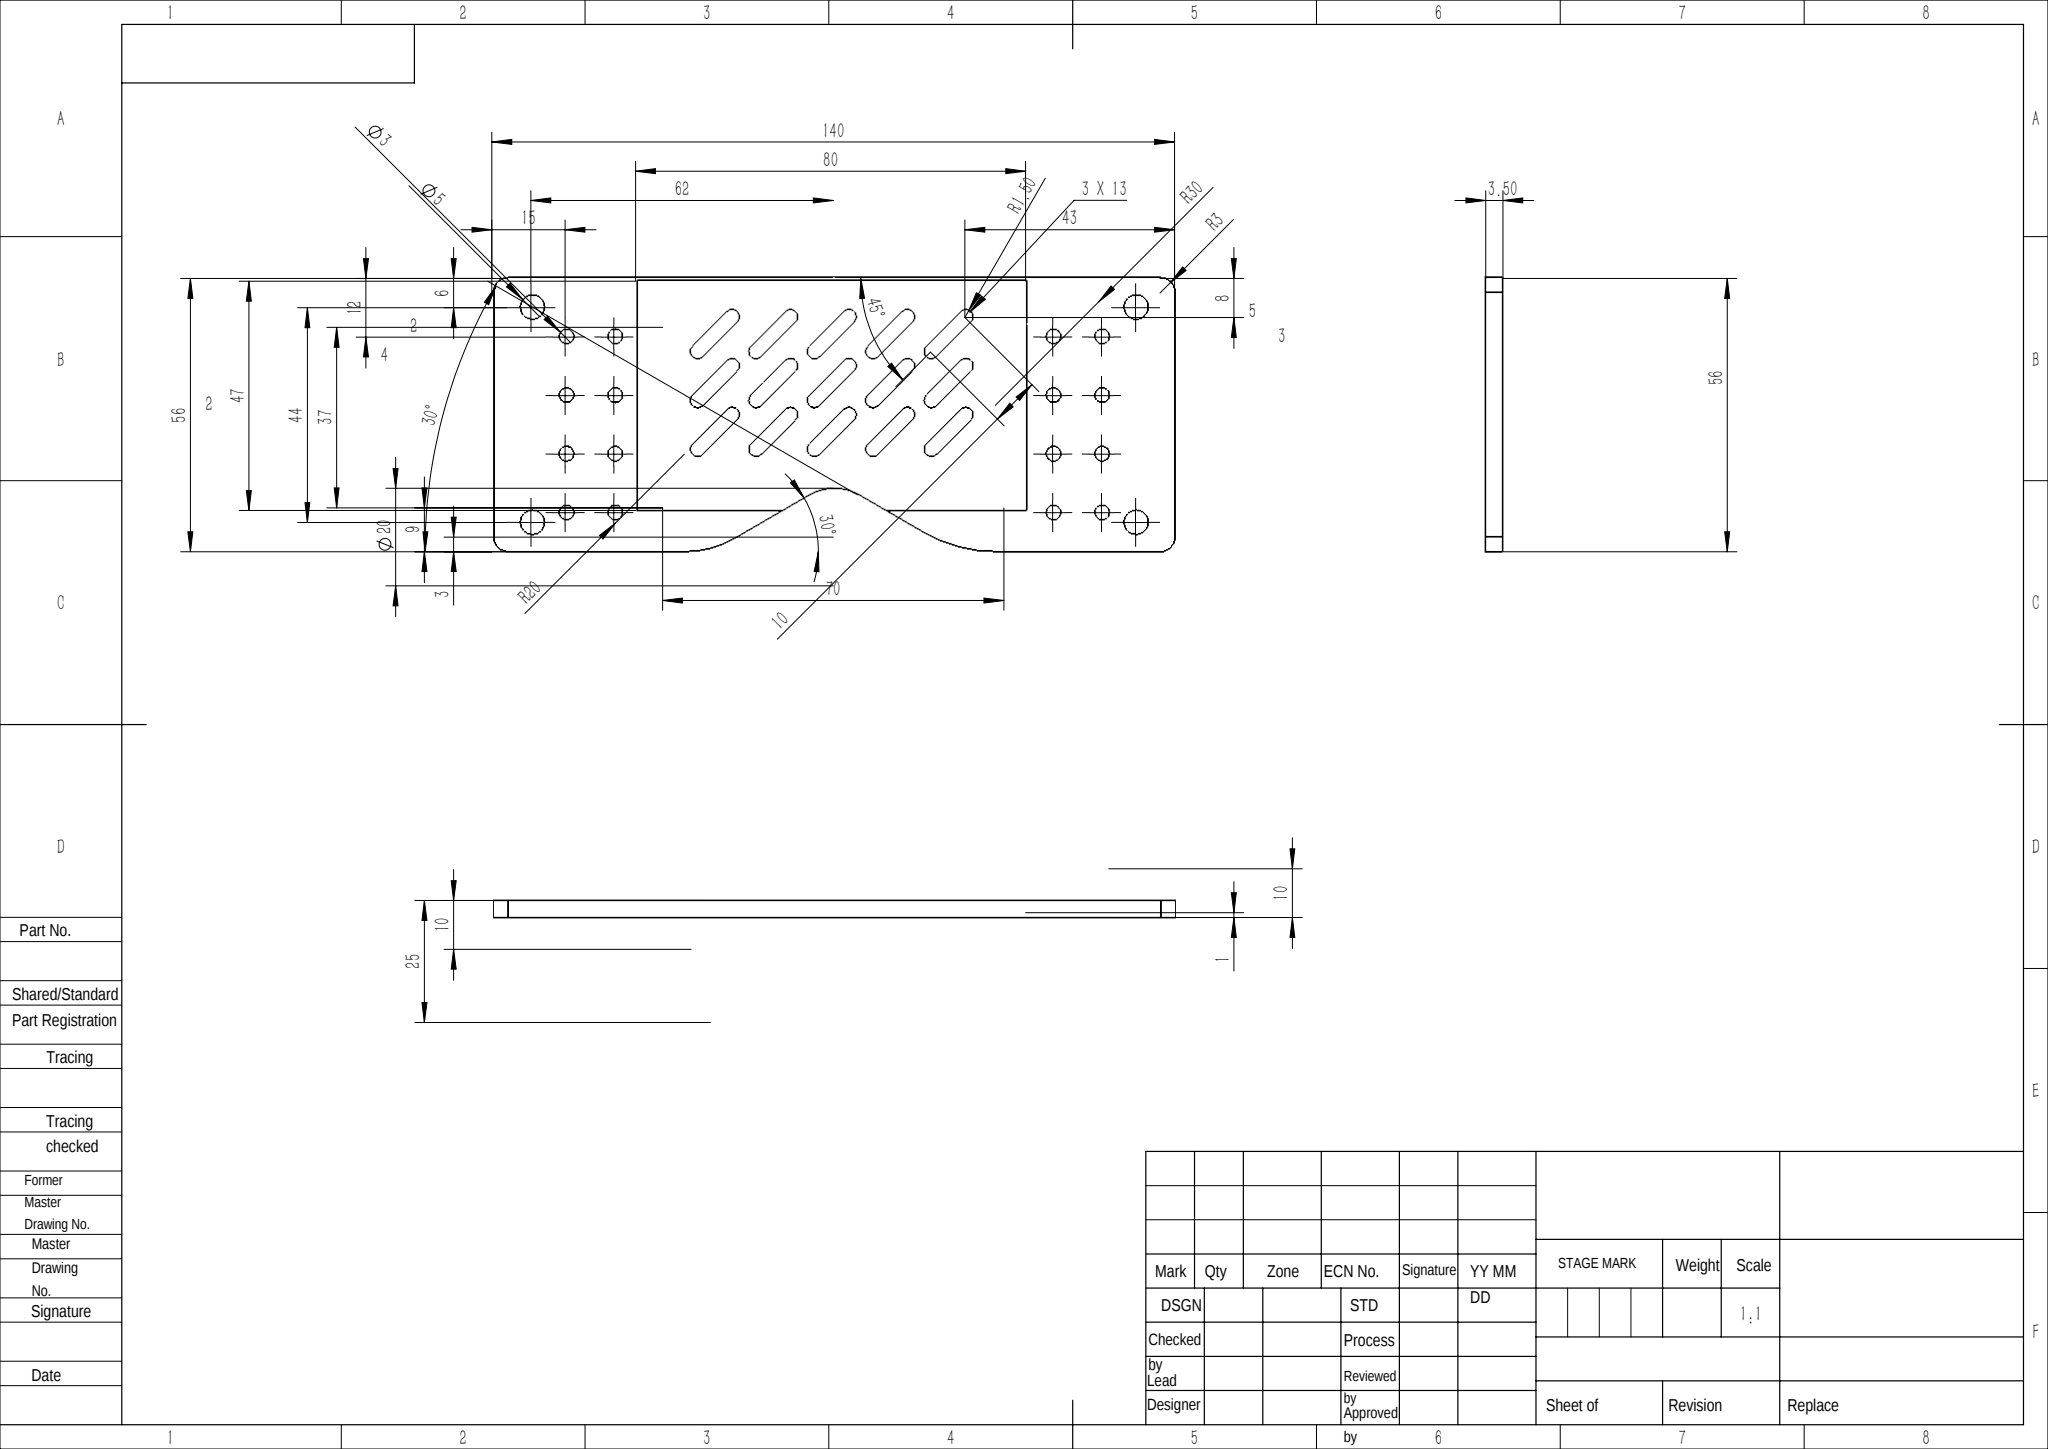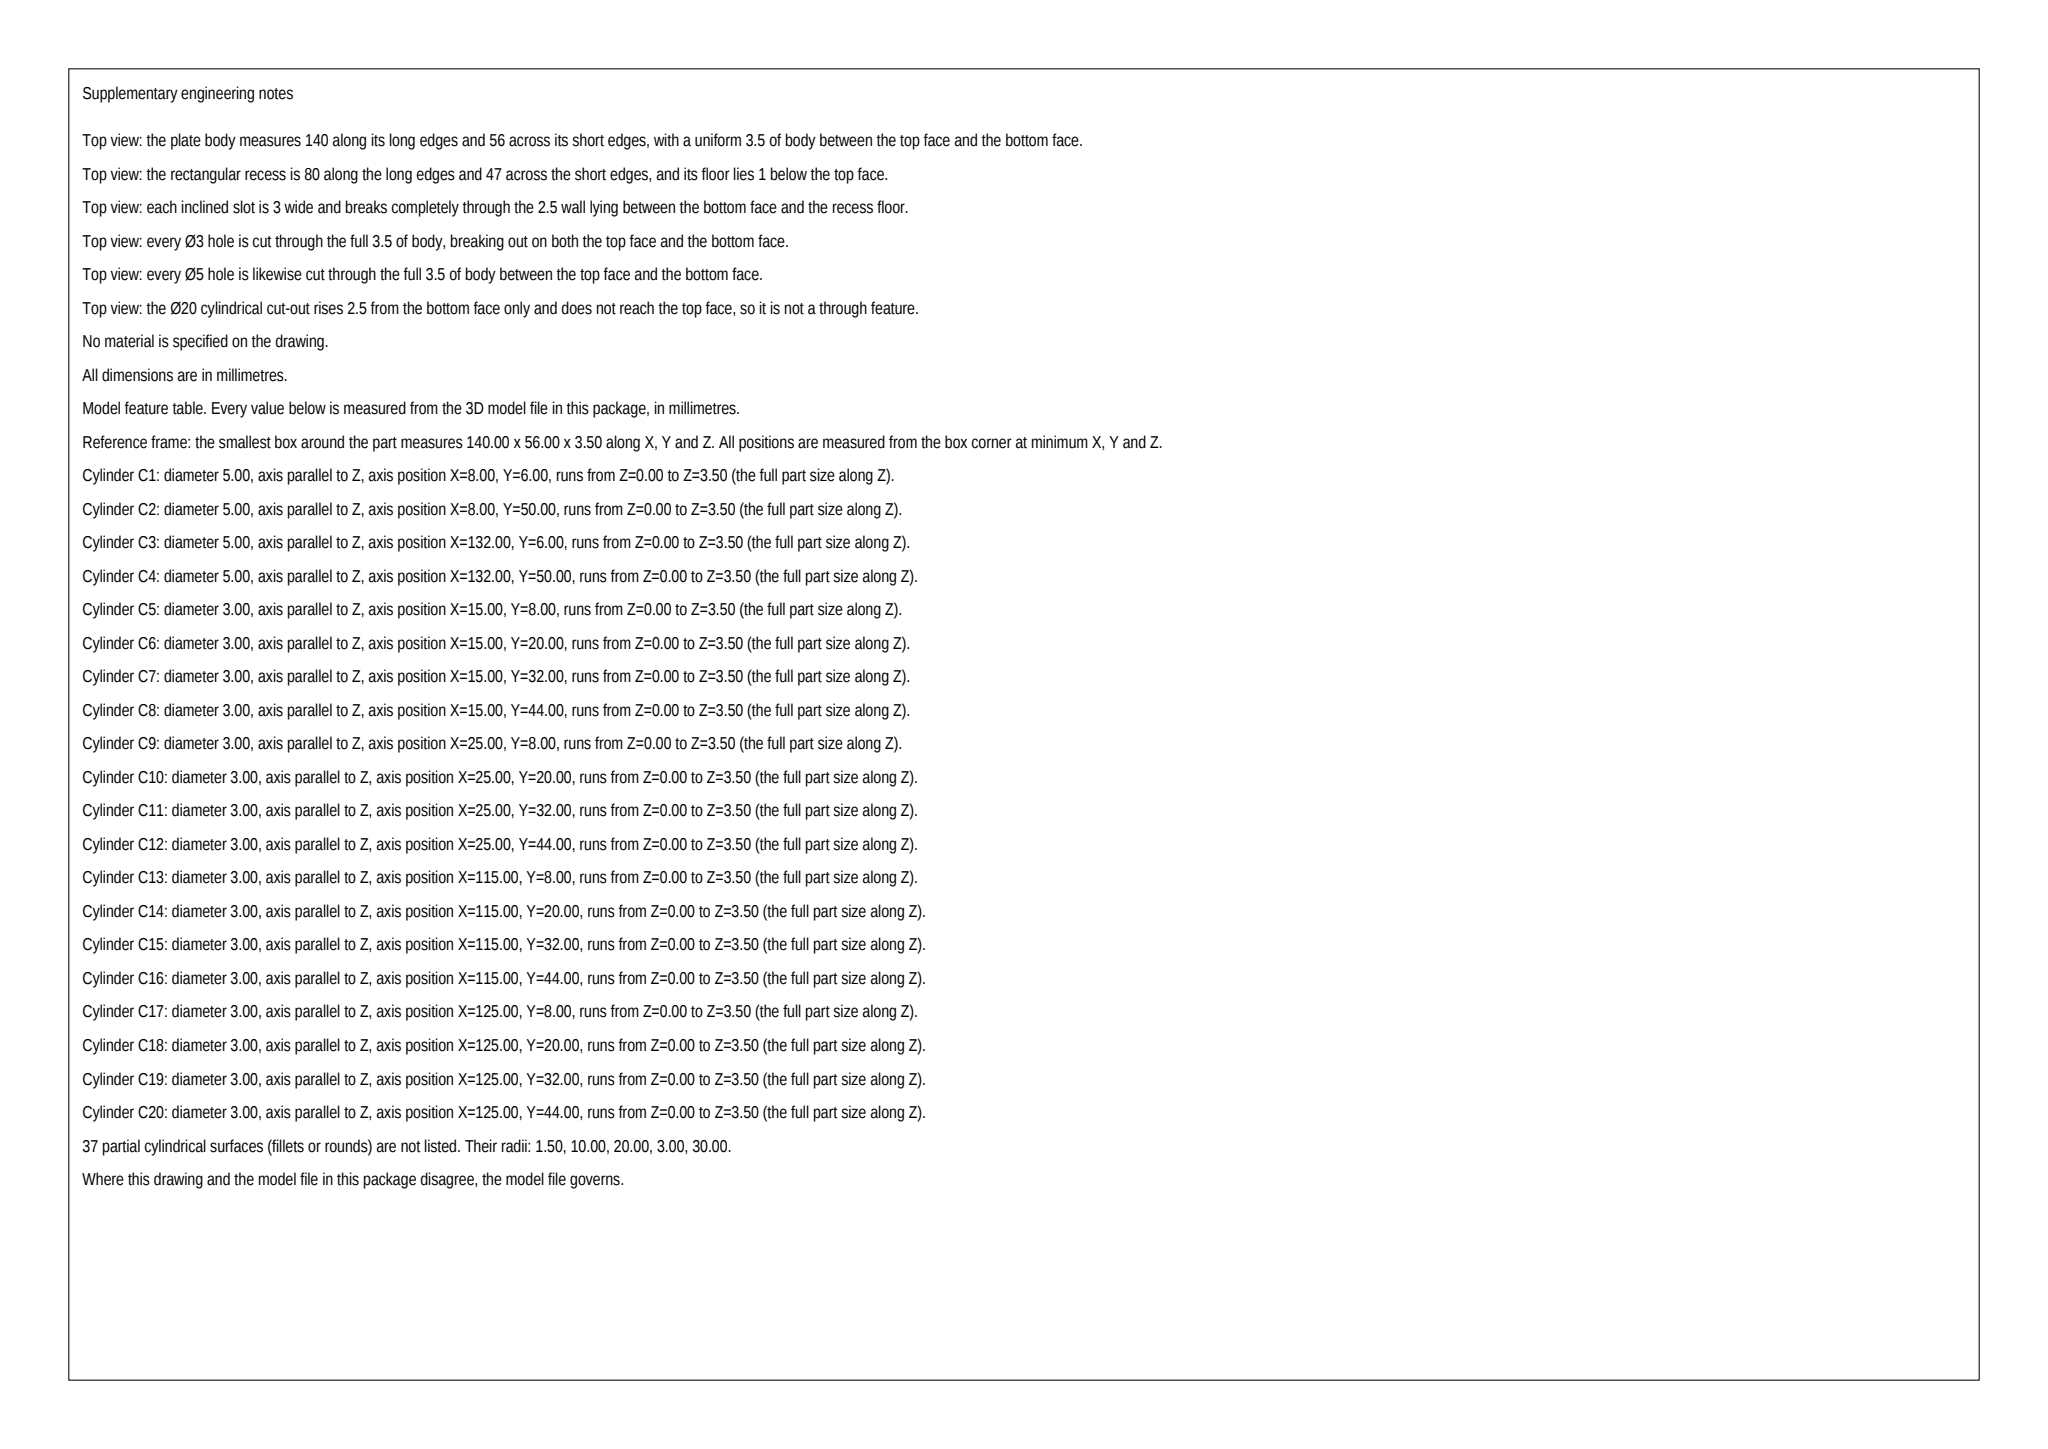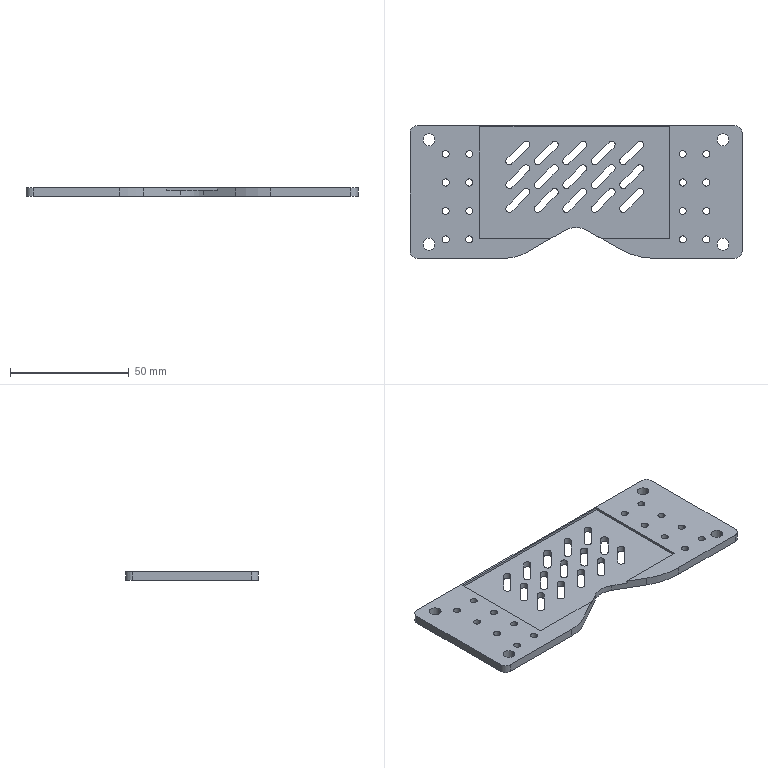Part | SolidWorks | mm | 1 solid | 137 faces | box 140 x 56 x 3.5 mm | volume 20359 mm3 | cylinder 92 | plane 45 | commonest cylinder face diameters 3 x77 5 x8 6 x4 20 x1 60 x1 40 x1
Drawing notes:
4X Ø6 THRU, CTRS 3 FROM EACH EDGE AT CORNERS | from the solid: dia 6 z-cyls at (3,3),(3,53),(137,3),(137,53), len 3.5 = full thk
Ø20 DP 2.5, CTR 70 FROM LH EDGE, 3 FROM BTM EDGE | from the solid: dia 20 z-cyl pos (70,3), length 2.5 in 3.5 plate
15X SLOT 3 X 13 DP 2.5, BLIND | from the solid: slot-end cyls dia 3 length 2.5; end ctr dist 10 => 13 OAL w/ R1.5
SLOT PATTERN 45°: 5 COL @12 PITCH X, 3 ROW @10 PITCH Y | from the solid: ends x=41.93,53.93,65.93,77.93,89.93; y=20.93,30.93,40.93; +7.07,+7.07 offset
16X Ø3 THRU; COL X=15,25,115,125; ROW Y=8,20,32,44 | from the solid: dia 3 len 3.5 cyls at listed x/y from bbox min corner
RH Ø3 COLS 25 & 15 FROM RH EDGE; 2X Ø5 8 FROM RH EDGE, Y=6 & 50 | from the solid: dia3 x=115,125 (140-25,140-15); dia5 x=132 (140-8), y=6,50
R20 CUT-OUT CTR X39.44 Y20; R30 CUT-OUT CTR X103.23 Y30 | from the solid: dia 40 cyl pos (39.44,20); dia 60 cyl pos (103.23,30)
POCKET FACES X29.46 & X109.46, Y8.45 & Y55.45 DP 2.5 | from the solid: planes x=29.46,109.46; y=8.45,55.45; z=2.5 floor
POCKET FLOOR Z2.5 FROM BTM: 1 THK WEB IN 3.5 PLATE | from the solid: z planes at 0, 2.5, 3.5
3X13 SLOT GRID: 1ST SLOT CTR 41.93 FROM LH EDGE, 20.93 FROM BTM | from the solid: slot cyl ctrs start at [41.93,20.93]; pitch 12 X, 10 Y; bbox 140x56 min corner datum
2X Ø5 THRU, 8 FROM LH EDGE, 6 & 50 FROM BTM EDGE | from the solid: cylinders dia 5 z-axis at [8,6] and [8,50], length 3.5 (thru 3.5 plate)
POCKET DP 1.0 FROM TOP FACE; FLOOR AT Z2.5 FROM BTM | from the solid: z planes at 0, 2.5, 3.5; floor plane z=2.5, top face z=3.5